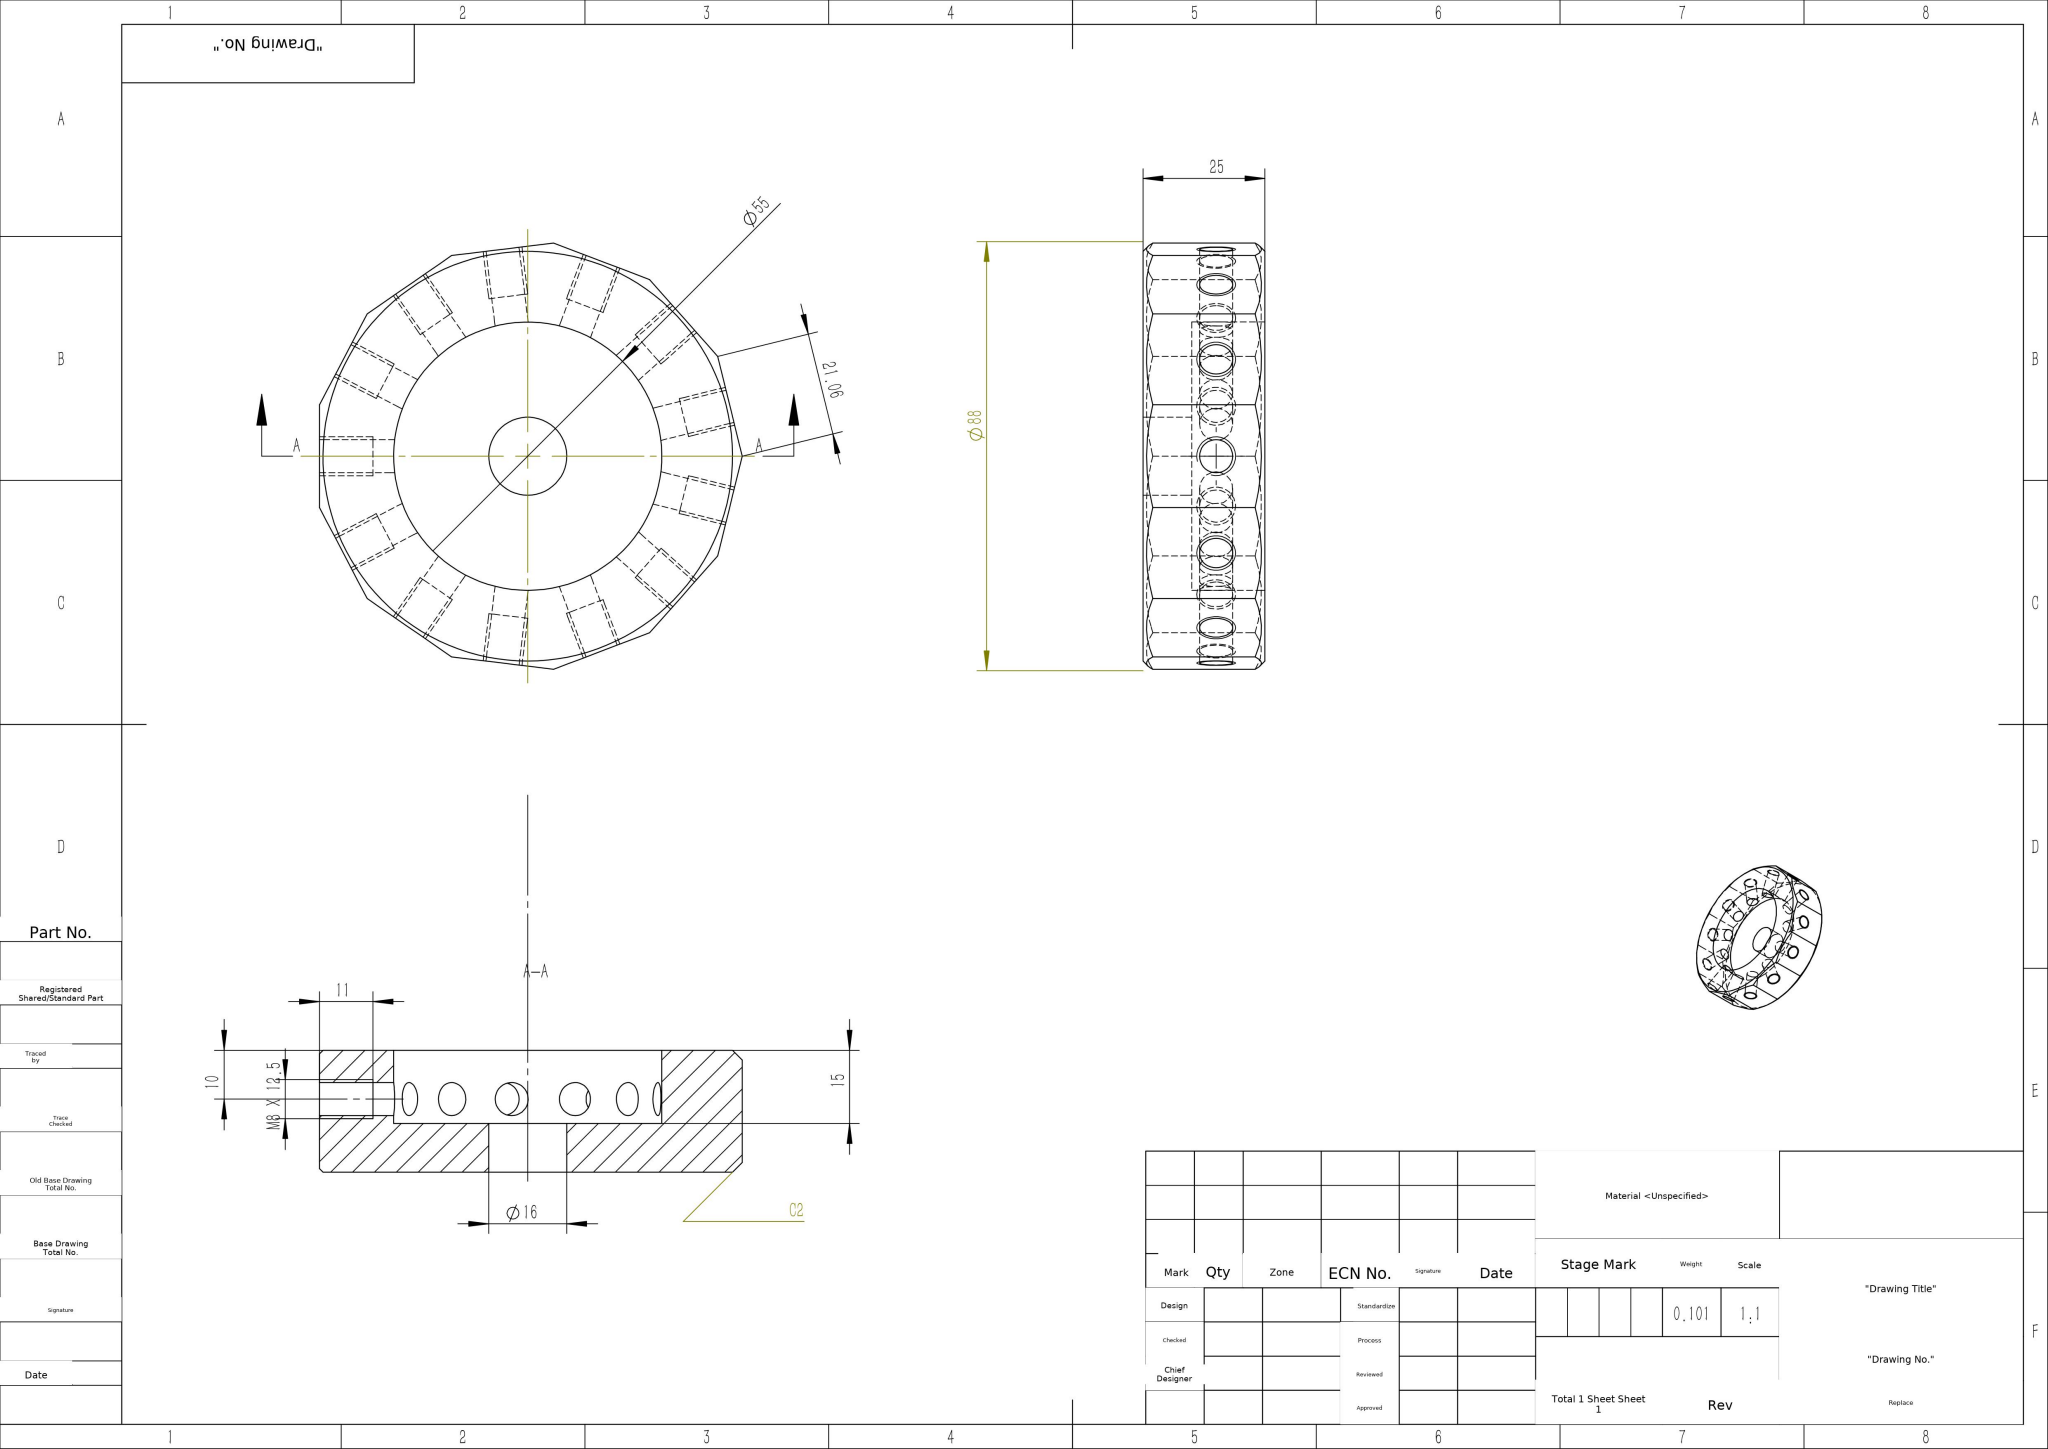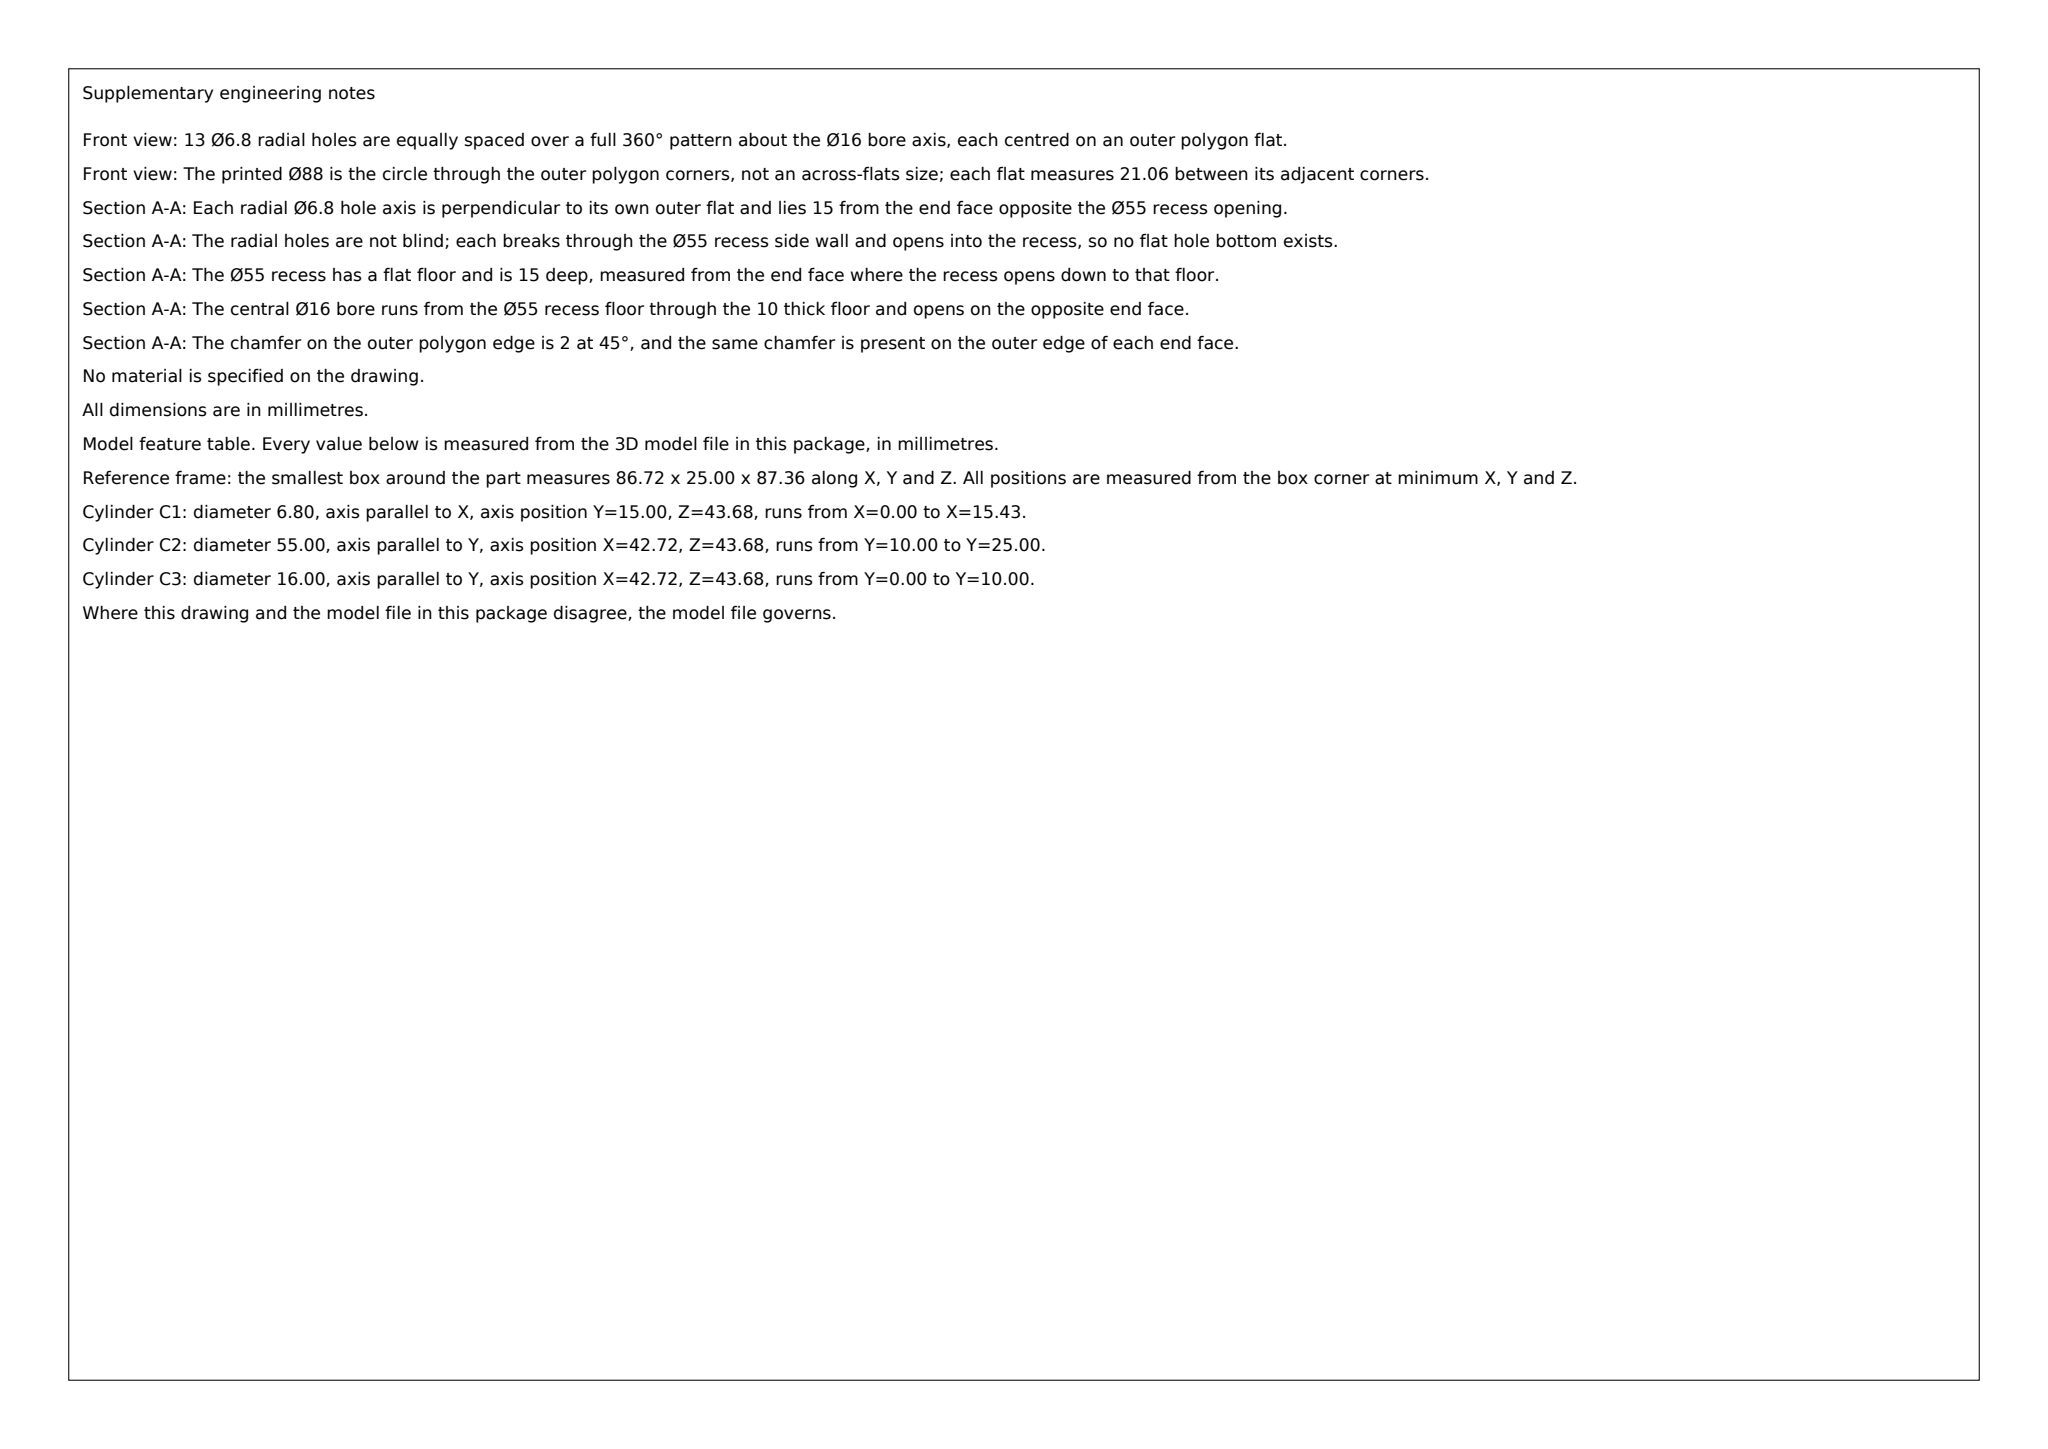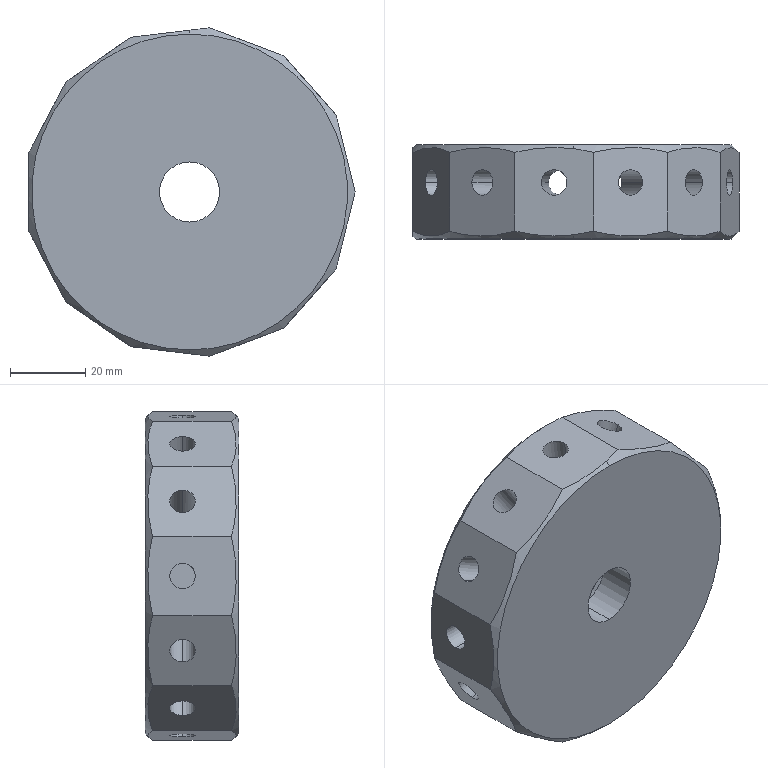Part | SolidWorks | mm | 1 solid | 50 faces | box 86.72 x 25 x 87.36 mm | volume 100950 mm3 | cylinder 30 | plane 16 | cone 4 | commonest cylinder face diameters 6.8 x26 16 x2 55 x2
Drawing notes:
13 X M8 x 12.5 RADIAL TAPPED HOLES, EQSP 27.69°, 1 PER FLAT | from the solid: 13 Ø6.8 radial cylinders, axes at y=15, one normal to each of 13 flats; 360/13=27.69°
TAP DRILL Ø6.8 DP 15.4 FROM FLAT, EA RADIAL HOLE | from the solid: Ø6.8 x-axis hole from x=1.3 (flat face plane x=1.3) to x=16.7 -> 15.4 deep
RADIAL HOLE AXES 15 FROM Ø16 END FACE, 10 FROM Ø55 FACE | from the solid: all Ø6.8 axes at y=15.0; Ø16 bore face y=0, Ø55 face y=25
13 FLATS EQSP 27.69°, 21.06 WIDE, Ø88 ACROSS CORNERS, 1 FLAT PERP A-A CL | from the solid: 12 inclined planes + plane x=1.3 = 13 flats; apothem 42.7 -> circumscribed Ø88; flat at x=1.3 normal to A-A hole axis
C2 (2 X 45°) ON Ø88 OUTER EDGE, BOTH END FACES | from the solid: 4 cones 90° incl, ref dia 88/84, y=0-2 and y=23-25, outer edge both faces
build123d program:
from build123d import *

# Parameters (mm, degrees)
SKETCH1_R           = 44
BOSS_EXTRUDE1_DEPTH = 25
SKETCH2_R           = 27.5
CUT_EXTRUDE1_DEPTH  = 15
SKETCH4_R           = 3.4
CUT_EXTRUDE2_DEPTH  = 50
CIRPATTERN1_COUNT   = 13
SKETCH5_R           = 8
CUT_EXTRUDE3_DEPTH  = 50
CHAMFER1_SIZE       = 2
SKETCH6_R           = 50.101
CUT_EXTRUDE6_DEPTH  = 50


with BuildPart() as part:
    # Sketch1 → Boss-Extrude1 (new body)
    with BuildSketch(Plane(origin=(0, 0, 0), x_dir=(1, 0, 0), z_dir=(0, 1, 0))):
        with Locations(Location((0, 0, 0), (0, 0, 270))):
            Circle(SKETCH1_R)
    extrude(amount=BOSS_EXTRUDE1_DEPTH)

    # Sketch2 → Cut-Extrude1 (cut)
    with BuildSketch(Plane(origin=(0, 25, 0), x_dir=(1, 0, 0), z_dir=(0, 1, 0))):
        with Locations(Location((0, 0, 0), (0, 0, 270))):
            Circle(SKETCH2_R)
    extrude(amount=-CUT_EXTRUDE1_DEPTH, mode=Mode.SUBTRACT)

    # Sketch4 → Cut-Extrude2 (cut)
    with BuildSketch(Plane.ZY.offset(44)):
        with Locations((0, 15)):
            Circle(SKETCH4_R)
    cut_extrude2 = extrude(amount=-CUT_EXTRUDE2_DEPTH, mode=Mode.SUBTRACT)

    # CirPattern1: Cut-Extrude2 ×13 about axis
    cirpattern1_axis = Axis((0, 25, 0), (0, -1, 0))
    for i in range(1, CIRPATTERN1_COUNT):
        add(cut_extrude2.rotate(cirpattern1_axis, i * 360 / CIRPATTERN1_COUNT), mode=Mode.SUBTRACT)

    # Sketch5 → Cut-Extrude3 (cut)
    with BuildSketch(Plane(origin=(0, 10, 0), x_dir=(1, 0, 0), z_dir=(0, 1, 0))):
        with Locations(Location((0, 0, 0), (0, 0, 270))):
            Circle(SKETCH5_R)
    extrude(amount=-CUT_EXTRUDE3_DEPTH, mode=Mode.SUBTRACT)

    # Chamfer1
    chamfer1_edges = [part.edges().sort_by_distance(p)[0] for p in [
        (0, 0, -44),
        (0, 25, -44),
    ]]
    chamfer(chamfer1_edges, length=CHAMFER1_SIZE)

    # Sketch6 → Cut-Extrude6 (cut)
    with BuildSketch(Plane(origin=(0, 25, 0), x_dir=(1, 0, 0), z_dir=(0, 1, 0))):
        Circle(SKETCH6_R)
        Polygon((24.995, 36.211), (5.304, 43.679), (-15.603, 41.141), (-32.934, 29.177), (-42.721, 10.53), (-42.721, -10.53), (-32.934, -29.177), (-15.603, -41.141), (5.304, -43.679), (24.995, -36.211), (38.96, -20.448), (44, 0), (38.96, 20.448), align=None, mode=Mode.SUBTRACT)
    extrude(amount=-CUT_EXTRUDE6_DEPTH, mode=Mode.SUBTRACT)


solid = part.part